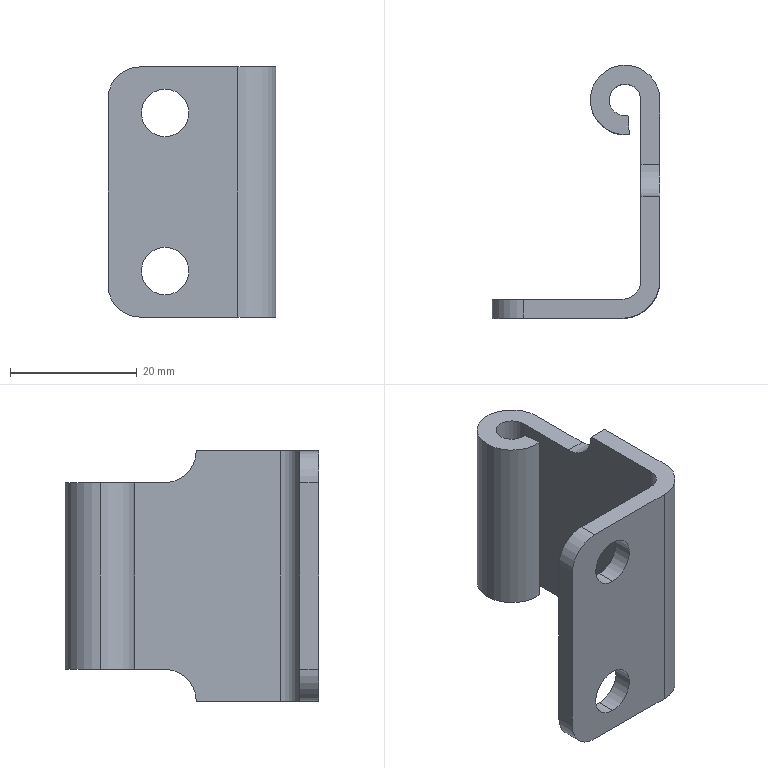Component | SolidWorks | Hinge1-1 | 1 solid | 24 faces | box 26.5 x 40 x 39.5 mm | volume 7641 mm3 | cylinder 14 | plane 10 | commonest cylinder face diameters 7.5 x4 10 x4 5 x2 11 x2 12 x1 6 x1
STEP:
#1=COLOUR_RGB('',0.7922,0.8196,0.9333);
#2=FILL_AREA_STYLE_COLOUR('',#1);
#3=FILL_AREA_STYLE('',(#2));
#4=SURFACE_STYLE_FILL_AREA(#3);
#5=SURFACE_SIDE_STYLE('',(#4));
#6=SURFACE_STYLE_USAGE(.BOTH.,#5);
#7=PRESENTATION_STYLE_ASSIGNMENT((#6));
#8=CARTESIAN_POINT('',(-50.116,6.946,101.261));
#9=VERTEX_POINT('',#8);
#10=CARTESIAN_POINT('',(-50.116,6.946,101.556));
#11=VERTEX_POINT('',#10);
#12=CARTESIAN_POINT('',(-50.116,6.946,101.408));
#13=DIRECTION('',(0.,1.,0.));
#14=DIRECTION('',(0.,0.,1.));
#15=AXIS2_PLACEMENT_3D('',#12,#13,#14);
#16=CIRCLE('',#15,0.1476);
#17=EDGE_CURVE('',#9,#11,#16,.T.);
#18=ORIENTED_EDGE('',*,*,#17,.F.);
#19=CARTESIAN_POINT('',(-50.116,7.064,101.261));
#20=VERTEX_POINT('',#19);
#21=CARTESIAN_POINT('',(-50.116,5.509,101.261));
#22=DIRECTION('',(0.,1.,0.));
#23=VECTOR('',#22,39.37);
#24=LINE('',#21,#23);
#25=EDGE_CURVE('',#9,#20,#24,.T.);
#26=ORIENTED_EDGE('',*,*,#25,.T.);
#27=CARTESIAN_POINT('',(-50.116,7.064,101.556));
#28=VERTEX_POINT('',#27);
#29=CARTESIAN_POINT('',(-50.116,7.064,101.408));
#30=DIRECTION('',(0.,1.,0.));
#31=DIRECTION('',(0.,0.,-1.));
#32=AXIS2_PLACEMENT_3D('',#29,#30,#31);
#33=CIRCLE('',#32,0.1476);
#34=EDGE_CURVE('',#20,#28,#33,.T.);
#35=ORIENTED_EDGE('',*,*,#34,.T.);
#36=CARTESIAN_POINT('',(-50.116,5.509,101.556));
#37=DIRECTION('',(0.,1.,0.));
#38=VECTOR('',#37,39.37);
#39=LINE('',#36,#38);
#40=EDGE_CURVE('',#11,#28,#39,.T.);
#41=ORIENTED_EDGE('',*,*,#40,.F.);
#42=EDGE_LOOP('',(#18,#26,#35,#41));
#43=FACE_OUTER_BOUND('',#42,.T.);
#44=CARTESIAN_POINT('',(-50.116,5.509,101.408));
#45=DIRECTION('',(0.,1.,0.));
#46=DIRECTION('',(0.,0.,1.));
#47=AXIS2_PLACEMENT_3D('',#44,#45,#46);
#48=CYLINDRICAL_SURFACE('',#47,0.1476);
#49=ADVANCED_FACE('',(#43),#48,.F.);
#50=CARTESIAN_POINT('',(-50.116,6.946,102.245));
#51=VERTEX_POINT('',#50);
#52=CARTESIAN_POINT('',(-50.116,6.946,102.54));
#53=VERTEX_POINT('',#52);
#54=CARTESIAN_POINT('',(-50.116,6.946,102.393));
#55=DIRECTION('',(0.,1.,0.));
#56=DIRECTION('',(0.,0.,1.));
#57=AXIS2_PLACEMENT_3D('',#54,#55,#56);
#58=CIRCLE('',#57,0.1476);
#59=EDGE_CURVE('',#51,#53,#58,.T.);
#60=ORIENTED_EDGE('',*,*,#59,.F.);
#61=CARTESIAN_POINT('',(-50.116,7.064,102.245));
#62=VERTEX_POINT('',#61);
#63=CARTESIAN_POINT('',(-50.116,5.509,102.245));
#64=DIRECTION('',(0.,1.,0.));
#65=VECTOR('',#64,39.37);
#66=LINE('',#63,#65);
#67=EDGE_CURVE('',#51,#62,#66,.T.);
#68=ORIENTED_EDGE('',*,*,#67,.T.);
#69=CARTESIAN_POINT('',(-50.116,7.064,102.54));
#70=VERTEX_POINT('',#69);
#71=CARTESIAN_POINT('',(-50.116,7.064,102.393));
#72=DIRECTION('',(0.,1.,0.));
#73=DIRECTION('',(0.,0.,1.));
#74=AXIS2_PLACEMENT_3D('',#71,#72,#73);
#75=CIRCLE('',#74,0.1476);
#76=EDGE_CURVE('',#62,#70,#75,.T.);
#77=ORIENTED_EDGE('',*,*,#76,.T.);
#78=CARTESIAN_POINT('',(-50.116,5.509,102.54));
#79=DIRECTION('',(0.,1.,0.));
#80=VECTOR('',#79,39.37);
#81=LINE('',#78,#80);
#82=EDGE_CURVE('',#53,#70,#81,.T.);
#83=ORIENTED_EDGE('',*,*,#82,.F.);
#84=EDGE_LOOP('',(#60,#68,#77,#83));
#85=FACE_OUTER_BOUND('',#84,.T.);
#86=CARTESIAN_POINT('',(-50.116,5.509,102.393));
#87=DIRECTION('',(0.,1.,0.));
#88=DIRECTION('',(0.,0.,1.));
#89=AXIS2_PLACEMENT_3D('',#86,#87,#88);
#90=CYLINDRICAL_SURFACE('',#89,0.1476);
#91=ADVANCED_FACE('',(#85),#90,.F.);
#92=CARTESIAN_POINT('',(-49.545,8.304,102.481));
#93=VERTEX_POINT('',#92);
#94=CARTESIAN_POINT('',(-49.742,8.304,102.481));
#95=VERTEX_POINT('',#94);
#96=CARTESIAN_POINT('',(-49.643,8.304,102.481));
#97=DIRECTION('',(0.,0.,1.));
#98=DIRECTION('',(-1.,0.,0.));
#99=AXIS2_PLACEMENT_3D('',#96,#97,#98);
#100=CIRCLE('',#99,0.09843);
#101=EDGE_CURVE('',#93,#95,#100,.T.);
#102=ORIENTED_EDGE('',*,*,#101,.T.);
#103=CARTESIAN_POINT('',(-49.742,8.304,101.32));
#104=VERTEX_POINT('',#103);
#105=CARTESIAN_POINT('',(-49.742,8.304,102.678));
#106=DIRECTION('',(0.,0.,-1.));
#107=VECTOR('',#106,39.37);
#108=LINE('',#105,#107);
#109=EDGE_CURVE('',#95,#104,#108,.T.);
#110=ORIENTED_EDGE('',*,*,#109,.T.);
#111=CARTESIAN_POINT('',(-49.545,8.304,101.32));
#112=VERTEX_POINT('',#111);
#113=CARTESIAN_POINT('',(-49.643,8.304,101.32));
#114=DIRECTION('',(0.,0.,-1.));
#115=DIRECTION('',(0.,-1.,0.));
#116=AXIS2_PLACEMENT_3D('',#113,#114,#115);
#117=CIRCLE('',#116,0.09843);
#118=EDGE_CURVE('',#104,#112,#117,.T.);
#119=ORIENTED_EDGE('',*,*,#118,.T.);
#120=CARTESIAN_POINT('',(-49.545,8.304,102.678));
#121=DIRECTION('',(0.,0.,-1.));
#122=VECTOR('',#121,39.37);
#123=LINE('',#120,#122);
#124=EDGE_CURVE('',#93,#112,#123,.T.);
#125=ORIENTED_EDGE('',*,*,#124,.F.);
#126=EDGE_LOOP('',(#102,#110,#119,#125));
#127=FACE_OUTER_BOUND('',#126,.T.);
#128=CARTESIAN_POINT('',(-49.643,8.304,102.678));
#129=DIRECTION('',(0.,0.,-1.));
#130=DIRECTION('',(-1.,0.,0.));
#131=AXIS2_PLACEMENT_3D('',#128,#129,#130);
#132=CYLINDRICAL_SURFACE('',#131,0.09843);
#133=ADVANCED_FACE('',(#127),#132,.F.);
#134=CARTESIAN_POINT('',(-49.617,8.089,102.481));
#135=VERTEX_POINT('',#134);
#136=CARTESIAN_POINT('',(-49.86,8.304,102.481));
#137=VERTEX_POINT('',#136);
#138=CARTESIAN_POINT('',(-49.643,8.304,102.481));
#139=DIRECTION('',(0.,0.,-1.));
#140=DIRECTION('',(-1.,0.,0.));
#141=AXIS2_PLACEMENT_3D('',#138,#139,#140);
#142=CIRCLE('',#141,0.2165);
#143=EDGE_CURVE('',#135,#137,#142,.T.);
#144=ORIENTED_EDGE('',*,*,#143,.T.);
#145=CARTESIAN_POINT('',(-49.86,8.304,101.32));
#146=VERTEX_POINT('',#145);
#147=CARTESIAN_POINT('',(-49.86,8.304,102.678));
#148=DIRECTION('',(0.,0.,-1.));
#149=VECTOR('',#148,39.37);
#150=LINE('',#147,#149);
#151=EDGE_CURVE('',#137,#146,#150,.T.);
#152=ORIENTED_EDGE('',*,*,#151,.T.);
#153=CARTESIAN_POINT('',(-49.617,8.089,101.32));
#154=VERTEX_POINT('',#153);
#155=CARTESIAN_POINT('',(-49.643,8.304,101.32));
#156=DIRECTION('',(0.,-0.,1.));
#157=DIRECTION('',(0.,-1.,0.));
#158=AXIS2_PLACEMENT_3D('',#155,#156,#157);
#159=CIRCLE('',#158,0.2165);
#160=EDGE_CURVE('',#146,#154,#159,.T.);
#161=ORIENTED_EDGE('',*,*,#160,.T.);
#162=CARTESIAN_POINT('',(-49.617,8.089,102.678));
#163=DIRECTION('',(0.,0.,-1.));
#164=VECTOR('',#163,39.37);
#165=LINE('',#162,#164);
#166=EDGE_CURVE('',#135,#154,#165,.T.);
#167=ORIENTED_EDGE('',*,*,#166,.F.);
#168=EDGE_LOOP('',(#144,#152,#161,#167));
#169=FACE_OUTER_BOUND('',#168,.T.);
#170=CARTESIAN_POINT('',(-49.643,8.304,102.678));
#171=DIRECTION('',(0.,0.,-1.));
#172=DIRECTION('',(-1.,0.,0.));
#173=AXIS2_PLACEMENT_3D('',#170,#171,#172);
#174=CYLINDRICAL_SURFACE('',#173,0.2165);
#175=ADVANCED_FACE('',(#169),#174,.T.);
#176=CARTESIAN_POINT('',(-50.47,7.064,102.481));
#177=VERTEX_POINT('',#176);
#178=CARTESIAN_POINT('',(-50.47,7.064,101.32));
#179=VERTEX_POINT('',#178);
#180=CARTESIAN_POINT('',(-50.47,7.064,102.678));
#181=DIRECTION('',(0.,0.,-1.));
#182=VECTOR('',#181,39.37);
#183=LINE('',#180,#182);
#184=EDGE_CURVE('',#177,#179,#183,.T.);
#185=ORIENTED_EDGE('',*,*,#184,.T.);
#186=CARTESIAN_POINT('',(-50.47,6.946,101.32));
#187=VERTEX_POINT('',#186);
#188=CARTESIAN_POINT('',(-50.47,6.946,101.32));
#189=DIRECTION('',(0.,-1.,0.));
#190=VECTOR('',#189,39.37);
#191=LINE('',#188,#190);
#192=EDGE_CURVE('',#179,#187,#191,.T.);
#193=ORIENTED_EDGE('',*,*,#192,.T.);
#194=CARTESIAN_POINT('',(-50.47,6.946,102.481));
#195=VERTEX_POINT('',#194);
#196=CARTESIAN_POINT('',(-50.47,6.946,102.678));
#197=DIRECTION('',(0.,0.,-1.));
#198=VECTOR('',#197,39.37);
#199=LINE('',#196,#198);
#200=EDGE_CURVE('',#195,#187,#199,.T.);
#201=ORIENTED_EDGE('',*,*,#200,.F.);
#202=CARTESIAN_POINT('',(-50.47,7.064,102.481));
#203=DIRECTION('',(0.,1.,0.));
#204=VECTOR('',#203,39.37);
#205=LINE('',#202,#204);
#206=EDGE_CURVE('',#195,#177,#205,.T.);
#207=ORIENTED_EDGE('',*,*,#206,.T.);
#208=EDGE_LOOP('',(#185,#193,#201,#207));
#209=FACE_OUTER_BOUND('',#208,.T.);
#210=CARTESIAN_POINT('',(-50.47,7.064,102.678));
#211=DIRECTION('',(1.,0.,0.));
#212=DIRECTION('',(0.,0.,-1.));
#213=AXIS2_PLACEMENT_3D('',#210,#211,#212);
#214=PLANE('',#213);
#215=ADVANCED_FACE('',(#209),#214,.F.);
#216=CARTESIAN_POINT('',(-50.116,6.946,101.408));
#217=DIRECTION('',(0.,1.,0.));
#218=DIRECTION('',(0.,0.,1.));
#219=AXIS2_PLACEMENT_3D('',#216,#217,#218);
#220=CIRCLE('',#219,0.1476);
#221=EDGE_CURVE('',#11,#9,#220,.T.);
#222=ORIENTED_EDGE('',*,*,#221,.T.);
#223=ORIENTED_EDGE('',*,*,#17,.T.);
#224=EDGE_LOOP('',(#222,#223));
#225=FACE_BOUND('',#224,.T.);
#226=CARTESIAN_POINT('',(-50.116,6.946,102.393));
#227=DIRECTION('',(0.,1.,0.));
#228=DIRECTION('',(0.,0.,1.));
#229=AXIS2_PLACEMENT_3D('',#226,#227,#228);
#230=CIRCLE('',#229,0.1476);
#231=EDGE_CURVE('',#53,#51,#230,.T.);
#232=ORIENTED_EDGE('',*,*,#231,.T.);
#233=ORIENTED_EDGE('',*,*,#59,.T.);
#234=EDGE_LOOP('',(#232,#233));
#235=FACE_BOUND('',#234,.T.);
#236=ORIENTED_EDGE('',*,*,#200,.T.);
#237=CARTESIAN_POINT('',(-50.273,6.946,101.123));
#238=VERTEX_POINT('',#237);
#239=CARTESIAN_POINT('',(-50.273,6.946,101.32));
#240=DIRECTION('',(0.,-1.,0.));
#241=DIRECTION('',(0.,0.,1.));
#242=AXIS2_PLACEMENT_3D('',#239,#240,#241);
#243=CIRCLE('',#242,0.1969);
#244=EDGE_CURVE('',#187,#238,#243,.T.);
#245=ORIENTED_EDGE('',*,*,#244,.T.);
#246=CARTESIAN_POINT('',(-49.663,6.946,101.123));
#247=VERTEX_POINT('',#246);
#248=CARTESIAN_POINT('',(-50.47,6.946,101.123));
#249=DIRECTION('',(1.,0.,0.));
#250=VECTOR('',#249,39.37);
#251=LINE('',#248,#250);
#252=EDGE_CURVE('',#238,#247,#251,.T.);
#253=ORIENTED_EDGE('',*,*,#252,.T.);
#254=CARTESIAN_POINT('',(-49.663,6.946,102.678));
#255=VERTEX_POINT('',#254);
#256=CARTESIAN_POINT('',(-49.663,6.946,102.678));
#257=DIRECTION('',(0.,0.,-1.));
#258=VECTOR('',#257,39.37);
#259=LINE('',#256,#258);
#260=EDGE_CURVE('',#255,#247,#259,.T.);
#261=ORIENTED_EDGE('',*,*,#260,.F.);
#262=CARTESIAN_POINT('',(-50.273,6.946,102.678));
#263=VERTEX_POINT('',#262);
#264=CARTESIAN_POINT('',(-50.47,6.946,102.678));
#265=DIRECTION('',(1.,0.,0.));
#266=VECTOR('',#265,39.37);
#267=LINE('',#264,#266);
#268=EDGE_CURVE('',#263,#255,#267,.T.);
#269=ORIENTED_EDGE('',*,*,#268,.F.);
#270=CARTESIAN_POINT('',(-50.273,6.946,102.481));
#271=DIRECTION('',(0.,-1.,0.));
#272=DIRECTION('',(0.,0.,1.));
#273=AXIS2_PLACEMENT_3D('',#270,#271,#272);
#274=CIRCLE('',#273,0.1969);
#275=EDGE_CURVE('',#263,#195,#274,.T.);
#276=ORIENTED_EDGE('',*,*,#275,.T.);
#277=EDGE_LOOP('',(#236,#245,#253,#261,#269,#276));
#278=FACE_OUTER_BOUND('',#277,.T.);
#279=CARTESIAN_POINT('',(-50.47,6.946,102.678));
#280=DIRECTION('',(0.,1.,0.));
#281=DIRECTION('',(0.,0.,1.));
#282=AXIS2_PLACEMENT_3D('',#279,#280,#281);
#283=PLANE('',#282);
#284=ADVANCED_FACE('',(#225,#235,#278),#283,.F.);
#285=CARTESIAN_POINT('',(-49.427,7.182,101.123));
#286=VERTEX_POINT('',#285);
#287=CARTESIAN_POINT('',(-49.663,7.182,101.123));
#288=DIRECTION('',(0.,0.,1.));
#289=DIRECTION('',(-1.,0.,0.));
#290=AXIS2_PLACEMENT_3D('',#287,#288,#289);
#291=CIRCLE('',#290,0.2362);
#292=EDGE_CURVE('',#247,#286,#291,.T.);
#293=ORIENTED_EDGE('',*,*,#292,.T.);
#294=CARTESIAN_POINT('',(-49.427,7.182,102.678));
#295=VERTEX_POINT('',#294);
#296=CARTESIAN_POINT('',(-49.427,7.182,102.678));
#297=DIRECTION('',(0.,0.,-1.));
#298=VECTOR('',#297,39.37);
#299=LINE('',#296,#298);
#300=EDGE_CURVE('',#295,#286,#299,.T.);
#301=ORIENTED_EDGE('',*,*,#300,.F.);
#302=CARTESIAN_POINT('',(-49.663,7.182,102.678));
#303=DIRECTION('',(0.,0.,1.));
#304=DIRECTION('',(-1.,0.,0.));
#305=AXIS2_PLACEMENT_3D('',#302,#303,#304);
#306=CIRCLE('',#305,0.2362);
#307=EDGE_CURVE('',#255,#295,#306,.T.);
#308=ORIENTED_EDGE('',*,*,#307,.F.);
#309=ORIENTED_EDGE('',*,*,#260,.T.);
#310=EDGE_LOOP('',(#293,#301,#308,#309));
#311=FACE_OUTER_BOUND('',#310,.T.);
#312=CARTESIAN_POINT('',(-49.663,7.182,102.678));
#313=DIRECTION('',(0.,0.,-1.));
#314=DIRECTION('',(-1.,0.,0.));
#315=AXIS2_PLACEMENT_3D('',#312,#313,#314);
#316=CYLINDRICAL_SURFACE('',#315,0.2362);
#317=ADVANCED_FACE('',(#311),#316,.T.);
#318=CARTESIAN_POINT('',(-49.427,7.705,101.123));
#319=VERTEX_POINT('',#318);
#320=CARTESIAN_POINT('',(-49.427,7.182,101.123));
#321=DIRECTION('',(0.,1.,0.));
#322=VECTOR('',#321,39.37);
#323=LINE('',#320,#322);
#324=EDGE_CURVE('',#286,#319,#323,.T.);
#325=ORIENTED_EDGE('',*,*,#324,.T.);
#326=CARTESIAN_POINT('',(-49.427,7.902,101.32));
#327=VERTEX_POINT('',#326);
#328=CARTESIAN_POINT('',(-49.427,7.902,101.123));
#329=DIRECTION('',(1.,0.,0.));
#330=DIRECTION('',(0.,0.,-1.));
#331=AXIS2_PLACEMENT_3D('',#328,#329,#330);
#332=CIRCLE('',#331,0.1969);
#333=EDGE_CURVE('',#327,#319,#332,.T.);
#334=ORIENTED_EDGE('',*,*,#333,.F.);
#335=CARTESIAN_POINT('',(-49.427,8.304,101.32));
#336=VERTEX_POINT('',#335);
#337=CARTESIAN_POINT('',(-49.427,8.54,101.32));
#338=DIRECTION('',(0.,-1.,-0.));
#339=VECTOR('',#338,39.37);
#340=LINE('',#337,#339);
#341=EDGE_CURVE('',#336,#327,#340,.T.);
#342=ORIENTED_EDGE('',*,*,#341,.F.);
#343=CARTESIAN_POINT('',(-49.427,8.304,102.481));
#344=VERTEX_POINT('',#343);
#345=CARTESIAN_POINT('',(-49.427,8.304,102.678));
#346=DIRECTION('',(0.,0.,-1.));
#347=VECTOR('',#346,39.37);
#348=LINE('',#345,#347);
#349=EDGE_CURVE('',#344,#336,#348,.T.);
#350=ORIENTED_EDGE('',*,*,#349,.F.);
#351=CARTESIAN_POINT('',(-49.427,7.902,102.481));
#352=VERTEX_POINT('',#351);
#353=CARTESIAN_POINT('',(-49.427,8.54,102.481));
#354=DIRECTION('',(0.,1.,0.));
#355=VECTOR('',#354,39.37);
#356=LINE('',#353,#355);
#357=EDGE_CURVE('',#352,#344,#356,.T.);
#358=ORIENTED_EDGE('',*,*,#357,.F.);
#359=CARTESIAN_POINT('',(-49.427,7.705,102.678));
#360=VERTEX_POINT('',#359);
#361=CARTESIAN_POINT('',(-49.427,7.902,102.678));
#362=DIRECTION('',(1.,0.,0.));
#363=DIRECTION('',(0.,0.,1.));
#364=AXIS2_PLACEMENT_3D('',#361,#362,#363);
#365=CIRCLE('',#364,0.1969);
#366=EDGE_CURVE('',#360,#352,#365,.T.);
#367=ORIENTED_EDGE('',*,*,#366,.F.);
#368=CARTESIAN_POINT('',(-49.427,7.182,102.678));
#369=DIRECTION('',(0.,1.,0.));
#370=VECTOR('',#369,39.37);
#371=LINE('',#368,#370);
#372=EDGE_CURVE('',#295,#360,#371,.T.);
#373=ORIENTED_EDGE('',*,*,#372,.F.);
#374=ORIENTED_EDGE('',*,*,#300,.T.);
#375=EDGE_LOOP('',(#325,#334,#342,#350,#358,#367,#373,#374));
#376=FACE_OUTER_BOUND('',#375,.T.);
#377=CARTESIAN_POINT('',(-49.427,7.182,102.678));
#378=DIRECTION('',(-1.,0.,0.));
#379=DIRECTION('',(0.,0.,1.));
#380=AXIS2_PLACEMENT_3D('',#377,#378,#379);
#381=PLANE('',#380);
#382=ADVANCED_FACE('',(#376),#381,.F.);
#383=ORIENTED_EDGE('',*,*,#151,.F.);
#384=CARTESIAN_POINT('',(-49.643,8.304,102.481));
#385=DIRECTION('',(0.,0.,-1.));
#386=DIRECTION('',(-1.,0.,0.));
#387=AXIS2_PLACEMENT_3D('',#384,#385,#386);
#388=CIRCLE('',#387,0.2165);
#389=EDGE_CURVE('',#137,#344,#388,.T.);
#390=ORIENTED_EDGE('',*,*,#389,.T.);
#391=ORIENTED_EDGE('',*,*,#349,.T.);
#392=CARTESIAN_POINT('',(-49.643,8.304,101.32));
#393=DIRECTION('',(0.,-0.,1.));
#394=DIRECTION('',(0.,-1.,0.));
#395=AXIS2_PLACEMENT_3D('',#392,#393,#394);
#396=CIRCLE('',#395,0.2165);
#397=EDGE_CURVE('',#336,#146,#396,.T.);
#398=ORIENTED_EDGE('',*,*,#397,.T.);
#399=EDGE_LOOP('',(#383,#390,#391,#398));
#400=FACE_OUTER_BOUND('',#399,.T.);
#401=CARTESIAN_POINT('',(-49.643,8.304,102.678));
#402=DIRECTION('',(0.,0.,-1.));
#403=DIRECTION('',(-1.,0.,0.));
#404=AXIS2_PLACEMENT_3D('',#401,#402,#403);
#405=CYLINDRICAL_SURFACE('',#404,0.2165);
#406=ADVANCED_FACE('',(#400),#405,.T.);
#407=ORIENTED_EDGE('',*,*,#166,.T.);
#408=CARTESIAN_POINT('',(-49.625,8.207,101.32));
#409=VERTEX_POINT('',#408);
#410=CARTESIAN_POINT('',(-49.625,8.207,101.32));
#411=DIRECTION('',(-0.07321,0.9973,0.));
#412=VECTOR('',#411,39.37);
#413=LINE('',#410,#412);
#414=EDGE_CURVE('',#154,#409,#413,.T.);
#415=ORIENTED_EDGE('',*,*,#414,.T.);
#416=CARTESIAN_POINT('',(-49.625,8.207,102.481));
#417=VERTEX_POINT('',#416);
#418=CARTESIAN_POINT('',(-49.625,8.207,102.678));
#419=DIRECTION('',(0.,0.,-1.));
#420=VECTOR('',#419,39.37);
#421=LINE('',#418,#420);
#422=EDGE_CURVE('',#417,#409,#421,.T.);
#423=ORIENTED_EDGE('',*,*,#422,.F.);
#424=CARTESIAN_POINT('',(-49.625,8.207,102.481));
#425=DIRECTION('',(0.07321,-0.9973,0.));
#426=VECTOR('',#425,39.37);
#427=LINE('',#424,#426);
#428=EDGE_CURVE('',#417,#135,#427,.T.);
#429=ORIENTED_EDGE('',*,*,#428,.T.);
#430=EDGE_LOOP('',(#407,#415,#423,#429));
#431=FACE_OUTER_BOUND('',#430,.T.);
#432=CARTESIAN_POINT('',(-49.625,8.207,102.678));
#433=DIRECTION('',(-0.9973,-0.07321,0.));
#434=DIRECTION('',(0.07321,-0.9973,0.));
#435=AXIS2_PLACEMENT_3D('',#432,#433,#434);
#436=PLANE('',#435);
#437=ADVANCED_FACE('',(#431),#436,.F.);
#438=ORIENTED_EDGE('',*,*,#109,.F.);
#439=CARTESIAN_POINT('',(-49.643,8.304,102.481));
#440=DIRECTION('',(0.,0.,1.));
#441=DIRECTION('',(-1.,0.,0.));
#442=AXIS2_PLACEMENT_3D('',#439,#440,#441);
#443=CIRCLE('',#442,0.09843);
#444=EDGE_CURVE('',#95,#417,#443,.T.);
#445=ORIENTED_EDGE('',*,*,#444,.T.);
#446=ORIENTED_EDGE('',*,*,#422,.T.);
#447=CARTESIAN_POINT('',(-49.643,8.304,101.32));
#448=DIRECTION('',(0.,0.,-1.));
#449=DIRECTION('',(0.,-1.,0.));
#450=AXIS2_PLACEMENT_3D('',#447,#448,#449);
#451=CIRCLE('',#450,0.09843);
#452=EDGE_CURVE('',#409,#104,#451,.T.);
#453=ORIENTED_EDGE('',*,*,#452,.T.);
#454=EDGE_LOOP('',(#438,#445,#446,#453));
#455=FACE_OUTER_BOUND('',#454,.T.);
#456=CARTESIAN_POINT('',(-49.643,8.304,102.678));
#457=DIRECTION('',(0.,0.,-1.));
#458=DIRECTION('',(-1.,0.,0.));
#459=AXIS2_PLACEMENT_3D('',#456,#457,#458);
#460=CYLINDRICAL_SURFACE('',#459,0.09843);
#461=ADVANCED_FACE('',(#455),#460,.F.);
#462=CARTESIAN_POINT('',(-49.545,7.902,101.32));
#463=VERTEX_POINT('',#462);
#464=CARTESIAN_POINT('',(-49.545,7.182,101.32));
#465=DIRECTION('',(0.,-1.,-0.));
#466=VECTOR('',#465,39.37);
#467=LINE('',#464,#466);
#468=EDGE_CURVE('',#112,#463,#467,.T.);
#469=ORIENTED_EDGE('',*,*,#468,.T.);
#470=CARTESIAN_POINT('',(-49.545,7.705,101.123));
#471=VERTEX_POINT('',#470);
#472=CARTESIAN_POINT('',(-49.545,7.902,101.123));
#473=DIRECTION('',(1.,0.,0.));
#474=DIRECTION('',(0.,0.,-1.));
#475=AXIS2_PLACEMENT_3D('',#472,#473,#474);
#476=CIRCLE('',#475,0.1969);
#477=EDGE_CURVE('',#463,#471,#476,.T.);
#478=ORIENTED_EDGE('',*,*,#477,.T.);
#479=CARTESIAN_POINT('',(-49.545,7.182,101.123));
#480=VERTEX_POINT('',#479);
#481=CARTESIAN_POINT('',(-49.545,7.182,101.123));
#482=DIRECTION('',(0.,-1.,0.));
#483=VECTOR('',#482,39.37);
#484=LINE('',#481,#483);
#485=EDGE_CURVE('',#471,#480,#484,.T.);
#486=ORIENTED_EDGE('',*,*,#485,.T.);
#487=CARTESIAN_POINT('',(-49.545,7.182,102.678));
#488=VERTEX_POINT('',#487);
#489=CARTESIAN_POINT('',(-49.545,7.182,102.678));
#490=DIRECTION('',(0.,0.,-1.));
#491=VECTOR('',#490,39.37);
#492=LINE('',#489,#491);
#493=EDGE_CURVE('',#488,#480,#492,.T.);
#494=ORIENTED_EDGE('',*,*,#493,.F.);
#495=CARTESIAN_POINT('',(-49.545,7.705,102.678));
#496=VERTEX_POINT('',#495);
#497=CARTESIAN_POINT('',(-49.545,7.182,102.678));
#498=DIRECTION('',(0.,-1.,0.));
#499=VECTOR('',#498,39.37);
#500=LINE('',#497,#499);
#501=EDGE_CURVE('',#496,#488,#500,.T.);
#502=ORIENTED_EDGE('',*,*,#501,.F.);
#503=CARTESIAN_POINT('',(-49.545,7.902,102.481));
#504=VERTEX_POINT('',#503);
#505=CARTESIAN_POINT('',(-49.545,7.902,102.678));
#506=DIRECTION('',(1.,0.,0.));
#507=DIRECTION('',(0.,0.,-1.));
#508=AXIS2_PLACEMENT_3D('',#505,#506,#507);
#509=CIRCLE('',#508,0.1969);
#510=EDGE_CURVE('',#496,#504,#509,.T.);
#511=ORIENTED_EDGE('',*,*,#510,.T.);
#512=CARTESIAN_POINT('',(-49.545,7.182,102.481));
#513=DIRECTION('',(0.,1.,0.));
#514=VECTOR('',#513,39.37);
#515=LINE('',#512,#514);
#516=EDGE_CURVE('',#504,#93,#515,.T.);
#517=ORIENTED_EDGE('',*,*,#516,.T.);
#518=ORIENTED_EDGE('',*,*,#124,.T.);
#519=EDGE_LOOP('',(#469,#478,#486,#494,#502,#511,#517,#518));
#520=FACE_OUTER_BOUND('',#519,.T.);
#521=CARTESIAN_POINT('',(-49.545,7.182,102.678));
#522=DIRECTION('',(1.,0.,0.));
#523=DIRECTION('',(0.,0.,-1.));
#524=AXIS2_PLACEMENT_3D('',#521,#522,#523);
#525=PLANE('',#524);
#526=ADVANCED_FACE('',(#520),#525,.F.);
#527=CARTESIAN_POINT('',(-49.663,7.064,101.123));
#528=VERTEX_POINT('',#527);
#529=CARTESIAN_POINT('',(-49.663,7.182,101.123));
#530=DIRECTION('',(0.,0.,-1.));
#531=DIRECTION('',(1.,0.,0.));
#532=AXIS2_PLACEMENT_3D('',#529,#530,#531);
#533=CIRCLE('',#532,0.1181);
#534=EDGE_CURVE('',#480,#528,#533,.T.);
#535=ORIENTED_EDGE('',*,*,#534,.T.);
#536=CARTESIAN_POINT('',(-49.663,7.064,102.678));
#537=VERTEX_POINT('',#536);
#538=CARTESIAN_POINT('',(-49.663,7.064,102.678));
#539=DIRECTION('',(0.,0.,-1.));
#540=VECTOR('',#539,39.37);
#541=LINE('',#538,#540);
#542=EDGE_CURVE('',#537,#528,#541,.T.);
#543=ORIENTED_EDGE('',*,*,#542,.F.);
#544=CARTESIAN_POINT('',(-49.663,7.182,102.678));
#545=DIRECTION('',(0.,0.,-1.));
#546=DIRECTION('',(1.,0.,0.));
#547=AXIS2_PLACEMENT_3D('',#544,#545,#546);
#548=CIRCLE('',#547,0.1181);
#549=EDGE_CURVE('',#488,#537,#548,.T.);
#550=ORIENTED_EDGE('',*,*,#549,.F.);
#551=ORIENTED_EDGE('',*,*,#493,.T.);
#552=EDGE_LOOP('',(#535,#543,#550,#551));
#553=FACE_OUTER_BOUND('',#552,.T.);
#554=CARTESIAN_POINT('',(-49.663,7.182,102.678));
#555=DIRECTION('',(0.,0.,-1.));
#556=DIRECTION('',(-1.,0.,0.));
#557=AXIS2_PLACEMENT_3D('',#554,#555,#556);
#558=CYLINDRICAL_SURFACE('',#557,0.1181);
#559=ADVANCED_FACE('',(#553),#558,.F.);
#560=CARTESIAN_POINT('',(-50.116,7.064,101.408));
#561=DIRECTION('',(0.,1.,0.));
#562=DIRECTION('',(0.,0.,-1.));
#563=AXIS2_PLACEMENT_3D('',#560,#561,#562);
#564=CIRCLE('',#563,0.1476);
#565=EDGE_CURVE('',#28,#20,#564,.T.);
#566=ORIENTED_EDGE('',*,*,#565,.F.);
#567=ORIENTED_EDGE('',*,*,#34,.F.);
#568=EDGE_LOOP('',(#566,#567));
#569=FACE_BOUND('',#568,.T.);
#570=CARTESIAN_POINT('',(-50.116,7.064,102.393));
#571=DIRECTION('',(0.,1.,0.));
#572=DIRECTION('',(0.,0.,1.));
#573=AXIS2_PLACEMENT_3D('',#570,#571,#572);
#574=CIRCLE('',#573,0.1476);
#575=EDGE_CURVE('',#70,#62,#574,.T.);
#576=ORIENTED_EDGE('',*,*,#575,.F.);
#577=ORIENTED_EDGE('',*,*,#76,.F.);
#578=EDGE_LOOP('',(#576,#577));
#579=FACE_BOUND('',#578,.T.);
#580=CARTESIAN_POINT('',(-50.273,7.064,101.123));
#581=VERTEX_POINT('',#580);
#582=CARTESIAN_POINT('',(-50.47,7.064,101.123));
#583=DIRECTION('',(-1.,0.,0.));
#584=VECTOR('',#583,39.37);
#585=LINE('',#582,#584);
#586=EDGE_CURVE('',#528,#581,#585,.T.);
#587=ORIENTED_EDGE('',*,*,#586,.T.);
#588=CARTESIAN_POINT('',(-50.273,7.064,101.32));
#589=DIRECTION('',(0.,1.,0.));
#590=DIRECTION('',(0.,0.,-1.));
#591=AXIS2_PLACEMENT_3D('',#588,#589,#590);
#592=CIRCLE('',#591,0.1969);
#593=EDGE_CURVE('',#581,#179,#592,.T.);
#594=ORIENTED_EDGE('',*,*,#593,.T.);
#595=ORIENTED_EDGE('',*,*,#184,.F.);
#596=CARTESIAN_POINT('',(-50.273,7.064,102.678));
#597=VERTEX_POINT('',#596);
#598=CARTESIAN_POINT('',(-50.273,7.064,102.481));
#599=DIRECTION('',(0.,1.,0.));
#600=DIRECTION('',(0.,0.,-1.));
#601=AXIS2_PLACEMENT_3D('',#598,#599,#600);
#602=CIRCLE('',#601,0.1969);
#603=EDGE_CURVE('',#177,#597,#602,.T.);
#604=ORIENTED_EDGE('',*,*,#603,.T.);
#605=CARTESIAN_POINT('',(-50.47,7.064,102.678));
#606=DIRECTION('',(-1.,0.,0.));
#607=VECTOR('',#606,39.37);
#608=LINE('',#605,#607);
#609=EDGE_CURVE('',#537,#597,#608,.T.);
#610=ORIENTED_EDGE('',*,*,#609,.F.);
#611=ORIENTED_EDGE('',*,*,#542,.T.);
#612=EDGE_LOOP('',(#587,#594,#595,#604,#610,#611));
#613=FACE_OUTER_BOUND('',#612,.T.);
#614=CARTESIAN_POINT('',(-50.47,7.064,102.678));
#615=DIRECTION('',(0.,-1.,0.));
#616=DIRECTION('',(0.,0.,-1.));
#617=AXIS2_PLACEMENT_3D('',#614,#615,#616);
#618=PLANE('',#617);
#619=ADVANCED_FACE('',(#569,#579,#613),#618,.F.);
#620=ORIENTED_EDGE('',*,*,#609,.T.);
#621=CARTESIAN_POINT('',(-50.273,7.182,102.678));
#622=DIRECTION('',(0.,-1.,0.));
#623=VECTOR('',#622,39.37);
#624=LINE('',#621,#623);
#625=EDGE_CURVE('',#597,#263,#624,.T.);
#626=ORIENTED_EDGE('',*,*,#625,.T.);
#627=ORIENTED_EDGE('',*,*,#268,.T.);
#628=ORIENTED_EDGE('',*,*,#307,.T.);
#629=ORIENTED_EDGE('',*,*,#372,.T.);
#630=CARTESIAN_POINT('',(-50.47,7.705,102.678));
#631=DIRECTION('',(-1.,0.,0.));
#632=VECTOR('',#631,39.37);
#633=LINE('',#630,#632);
#634=EDGE_CURVE('',#360,#496,#633,.T.);
#635=ORIENTED_EDGE('',*,*,#634,.T.);
#636=ORIENTED_EDGE('',*,*,#501,.T.);
#637=ORIENTED_EDGE('',*,*,#549,.T.);
#638=EDGE_LOOP('',(#620,#626,#627,#628,#629,#635,#636,#637));
#639=FACE_OUTER_BOUND('',#638,.T.);
#640=CARTESIAN_POINT('',(-49.663,7.182,102.678));
#641=DIRECTION('',(0.,0.,-1.));
#642=DIRECTION('',(-1.,0.,0.));
#643=AXIS2_PLACEMENT_3D('',#640,#641,#642);
#644=PLANE('',#643);
#645=ADVANCED_FACE('',(#639),#644,.F.);
#646=ORIENTED_EDGE('',*,*,#252,.F.);
#647=CARTESIAN_POINT('',(-50.273,7.064,101.123));
#648=DIRECTION('',(0.,1.,0.));
#649=VECTOR('',#648,39.37);
#650=LINE('',#647,#649);
#651=EDGE_CURVE('',#238,#581,#650,.T.);
#652=ORIENTED_EDGE('',*,*,#651,.T.);
#653=ORIENTED_EDGE('',*,*,#586,.F.);
#654=ORIENTED_EDGE('',*,*,#534,.F.);
#655=ORIENTED_EDGE('',*,*,#485,.F.);
#656=CARTESIAN_POINT('',(-50.47,7.705,101.123));
#657=DIRECTION('',(-1.,0.,0.));
#658=VECTOR('',#657,39.37);
#659=LINE('',#656,#658);
#660=EDGE_CURVE('',#319,#471,#659,.T.);
#661=ORIENTED_EDGE('',*,*,#660,.F.);
#662=ORIENTED_EDGE('',*,*,#324,.F.);
#663=ORIENTED_EDGE('',*,*,#292,.F.);
#664=EDGE_LOOP('',(#646,#652,#653,#654,#655,#661,#662,#663));
#665=FACE_OUTER_BOUND('',#664,.T.);
#666=CARTESIAN_POINT('',(-49.663,7.182,101.123));
#667=DIRECTION('',(0.,0.,-1.));
#668=DIRECTION('',(-1.,0.,0.));
#669=AXIS2_PLACEMENT_3D('',#666,#667,#668);
#670=PLANE('',#669);
#671=ADVANCED_FACE('',(#665),#670,.T.);
#672=ORIENTED_EDGE('',*,*,#428,.F.);
#673=ORIENTED_EDGE('',*,*,#444,.F.);
#674=ORIENTED_EDGE('',*,*,#101,.F.);
#675=ORIENTED_EDGE('',*,*,#516,.F.);
#676=CARTESIAN_POINT('',(-50.47,7.902,102.481));
#677=DIRECTION('',(1.,0.,0.));
#678=VECTOR('',#677,39.37);
#679=LINE('',#676,#678);
#680=EDGE_CURVE('',#504,#352,#679,.T.);
#681=ORIENTED_EDGE('',*,*,#680,.T.);
#682=ORIENTED_EDGE('',*,*,#357,.T.);
#683=ORIENTED_EDGE('',*,*,#389,.F.);
#684=ORIENTED_EDGE('',*,*,#143,.F.);
#685=EDGE_LOOP('',(#672,#673,#674,#675,#681,#682,#683,#684));
#686=FACE_OUTER_BOUND('',#685,.T.);
#687=CARTESIAN_POINT('',(-50.47,8.54,102.481));
#688=DIRECTION('',(0.,0.,-1.));
#689=DIRECTION('',(-1.,0.,0.));
#690=AXIS2_PLACEMENT_3D('',#687,#688,#689);
#691=PLANE('',#690);
#692=ADVANCED_FACE('',(#686),#691,.F.);
#693=ORIENTED_EDGE('',*,*,#634,.F.);
#694=ORIENTED_EDGE('',*,*,#366,.T.);
#695=ORIENTED_EDGE('',*,*,#680,.F.);
#696=ORIENTED_EDGE('',*,*,#510,.F.);
#697=EDGE_LOOP('',(#693,#694,#695,#696));
#698=FACE_OUTER_BOUND('',#697,.T.);
#699=CARTESIAN_POINT('',(-50.47,7.902,102.678));
#700=DIRECTION('',(1.,0.,0.));
#701=DIRECTION('',(0.,0.,-1.));
#702=AXIS2_PLACEMENT_3D('',#699,#700,#701);
#703=CYLINDRICAL_SURFACE('',#702,0.1969);
#704=ADVANCED_FACE('',(#698),#703,.F.);
#705=ORIENTED_EDGE('',*,*,#341,.T.);
#706=CARTESIAN_POINT('',(-50.47,7.902,101.32));
#707=DIRECTION('',(1.,0.,0.));
#708=VECTOR('',#707,39.37);
#709=LINE('',#706,#708);
#710=EDGE_CURVE('',#463,#327,#709,.T.);
#711=ORIENTED_EDGE('',*,*,#710,.F.);
#712=ORIENTED_EDGE('',*,*,#468,.F.);
#713=ORIENTED_EDGE('',*,*,#118,.F.);
#714=ORIENTED_EDGE('',*,*,#452,.F.);
#715=ORIENTED_EDGE('',*,*,#414,.F.);
#716=ORIENTED_EDGE('',*,*,#160,.F.);
#717=ORIENTED_EDGE('',*,*,#397,.F.);
#718=EDGE_LOOP('',(#705,#711,#712,#713,#714,#715,#716,#717));
#719=FACE_OUTER_BOUND('',#718,.T.);
#720=CARTESIAN_POINT('',(-50.47,8.54,101.32));
#721=DIRECTION('',(0.,-0.,1.));
#722=DIRECTION('',(0.,-1.,-0.));
#723=AXIS2_PLACEMENT_3D('',#720,#721,#722);
#724=PLANE('',#723);
#725=ADVANCED_FACE('',(#719),#724,.F.);
#726=ORIENTED_EDGE('',*,*,#710,.T.);
#727=ORIENTED_EDGE('',*,*,#333,.T.);
#728=ORIENTED_EDGE('',*,*,#660,.T.);
#729=ORIENTED_EDGE('',*,*,#477,.F.);
#730=EDGE_LOOP('',(#726,#727,#728,#729));
#731=FACE_OUTER_BOUND('',#730,.T.);
#732=CARTESIAN_POINT('',(-50.47,7.902,101.123));
#733=DIRECTION('',(1.,0.,0.));
#734=DIRECTION('',(0.,0.,-1.));
#735=AXIS2_PLACEMENT_3D('',#732,#733,#734);
#736=CYLINDRICAL_SURFACE('',#735,0.1969);
#737=ADVANCED_FACE('',(#731),#736,.F.);
#738=ORIENTED_EDGE('',*,*,#593,.F.);
#739=ORIENTED_EDGE('',*,*,#651,.F.);
#740=ORIENTED_EDGE('',*,*,#244,.F.);
#741=ORIENTED_EDGE('',*,*,#192,.F.);
#742=EDGE_LOOP('',(#738,#739,#740,#741));
#743=FACE_OUTER_BOUND('',#742,.T.);
#744=CARTESIAN_POINT('',(-50.273,7.064,101.32));
#745=DIRECTION('',(0.,1.,0.));
#746=DIRECTION('',(0.,0.,1.));
#747=AXIS2_PLACEMENT_3D('',#744,#745,#746);
#748=CYLINDRICAL_SURFACE('',#747,0.1969);
#749=ADVANCED_FACE('',(#743),#748,.T.);
#750=ORIENTED_EDGE('',*,*,#603,.F.);
#751=ORIENTED_EDGE('',*,*,#206,.F.);
#752=ORIENTED_EDGE('',*,*,#275,.F.);
#753=ORIENTED_EDGE('',*,*,#625,.F.);
#754=EDGE_LOOP('',(#750,#751,#752,#753));
#755=FACE_OUTER_BOUND('',#754,.T.);
#756=CARTESIAN_POINT('',(-50.273,7.182,102.481));
#757=DIRECTION('',(0.,-1.,0.));
#758=DIRECTION('',(0.,0.,-1.));
#759=AXIS2_PLACEMENT_3D('',#756,#757,#758);
#760=CYLINDRICAL_SURFACE('',#759,0.1969);
#761=ADVANCED_FACE('',(#755),#760,.T.);
#762=ORIENTED_EDGE('',*,*,#67,.F.);
#763=ORIENTED_EDGE('',*,*,#231,.F.);
#764=ORIENTED_EDGE('',*,*,#82,.T.);
#765=ORIENTED_EDGE('',*,*,#575,.T.);
#766=EDGE_LOOP('',(#762,#763,#764,#765));
#767=FACE_OUTER_BOUND('',#766,.T.);
#768=CARTESIAN_POINT('',(-50.116,5.509,102.393));
#769=DIRECTION('',(0.,1.,0.));
#770=DIRECTION('',(0.,0.,1.));
#771=AXIS2_PLACEMENT_3D('',#768,#769,#770);
#772=CYLINDRICAL_SURFACE('',#771,0.1476);
#773=ADVANCED_FACE('',(#767),#772,.F.);
#774=ORIENTED_EDGE('',*,*,#25,.F.);
#775=ORIENTED_EDGE('',*,*,#221,.F.);
#776=ORIENTED_EDGE('',*,*,#40,.T.);
#777=ORIENTED_EDGE('',*,*,#565,.T.);
#778=EDGE_LOOP('',(#774,#775,#776,#777));
#779=FACE_OUTER_BOUND('',#778,.T.);
#780=CARTESIAN_POINT('',(-50.116,5.509,101.408));
#781=DIRECTION('',(0.,1.,0.));
#782=DIRECTION('',(0.,0.,1.));
#783=AXIS2_PLACEMENT_3D('',#780,#781,#782);
#784=CYLINDRICAL_SURFACE('',#783,0.1476);
#785=ADVANCED_FACE('',(#779),#784,.F.);
#786=CLOSED_SHELL('',(#49,#91,#133,#175,#215,#284,#317,#382,#406,#437,#461,#526,#559,#619,#645,#671,#692,#704,#725,#737,#749,#761,#773,#785));
#787=MANIFOLD_SOLID_BREP('',#786);
#788=STYLED_ITEM('',(#7),#787);
#789=PRESENTATION_LAYER_ASSIGNMENT('','',(#788));
#790=(LENGTH_UNIT()NAMED_UNIT(*)SI_UNIT($,.METRE.));
#791=LENGTH_MEASURE_WITH_UNIT(LENGTH_MEASURE(0.0254),#790);
#792=DIMENSIONAL_EXPONENTS(1.,0.,0.,0.,0.,0.,0.);
#793=(CONVERSION_BASED_UNIT('',#791)LENGTH_UNIT()NAMED_UNIT(#792));
#794=UNCERTAINTY_MEASURE_WITH_UNIT(LENGTH_MEASURE(0.00001),#793,'','');
#795=(NAMED_UNIT(*)PLANE_ANGLE_UNIT()SI_UNIT($,.RADIAN.));
#796=(NAMED_UNIT(*)SI_UNIT($,.STERADIAN.)SOLID_ANGLE_UNIT());
#797=(GEOMETRIC_REPRESENTATION_CONTEXT(3)GLOBAL_UNCERTAINTY_ASSIGNED_CONTEXT((#794))GLOBAL_UNIT_ASSIGNED_CONTEXT((#793,#795,#796))REPRESENTATION_CONTEXT('',''));
#798=MECHANICAL_DESIGN_GEOMETRIC_PRESENTATION_REPRESENTATION('',(#788),#797);
#799=CARTESIAN_POINT('',(0.,0.,0.));
#800=DIRECTION('',(0.,0.,1.));
#801=DIRECTION('',(1.,0.,0.));
#802=AXIS2_PLACEMENT_3D('',#799,#800,#801);
#803=(LENGTH_UNIT()NAMED_UNIT(*)SI_UNIT($,.METRE.));
#804=LENGTH_MEASURE_WITH_UNIT(LENGTH_MEASURE(0.0254),#803);
#805=DIMENSIONAL_EXPONENTS(1.,0.,0.,0.,0.,0.,0.);
#806=(CONVERSION_BASED_UNIT('',#804)LENGTH_UNIT()NAMED_UNIT(#805));
#807=UNCERTAINTY_MEASURE_WITH_UNIT(LENGTH_MEASURE(0.00001),#806,'','');
#808=(NAMED_UNIT(*)PLANE_ANGLE_UNIT()SI_UNIT($,.RADIAN.));
#809=(NAMED_UNIT(*)SI_UNIT($,.STERADIAN.)SOLID_ANGLE_UNIT());
#810=(GEOMETRIC_REPRESENTATION_CONTEXT(3)GLOBAL_UNCERTAINTY_ASSIGNED_CONTEXT((#807))GLOBAL_UNIT_ASSIGNED_CONTEXT((#806,#808,#809))REPRESENTATION_CONTEXT('',''));
#811=ADVANCED_BREP_SHAPE_REPRESENTATION('',(#787,#802),#810);